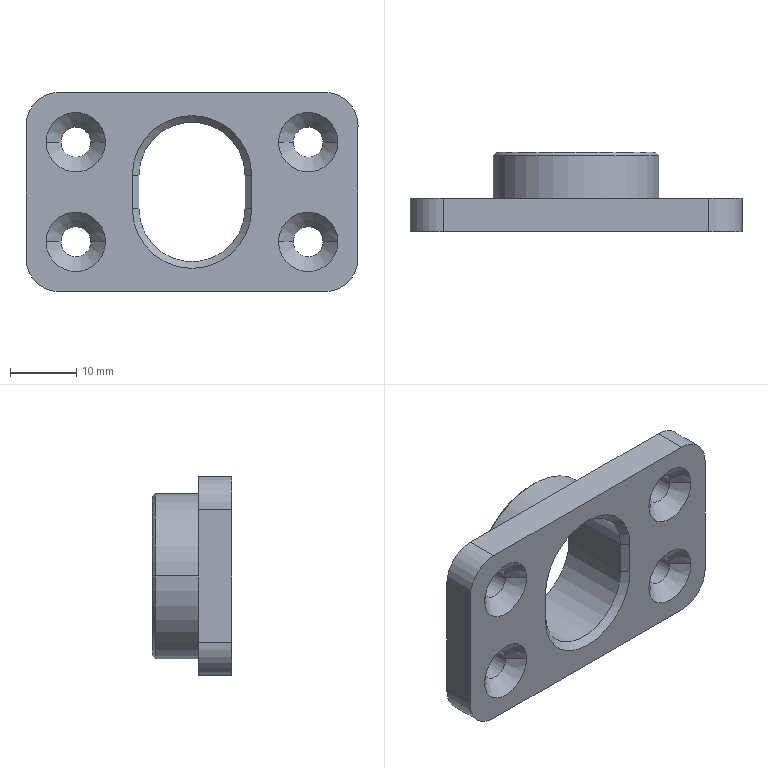Component | SolidWorks | MA060.03.03-08-1 | 1 solid | 39 faces | box 50 x 12 x 30 mm | volume 6910 mm3 | cylinder 16 | cone 12 | plane 11 | commonest cylinder face diameters 4.5 x8 10 x4 25 x2 16 x2 | material H68
build123d program:
from build123d import *

# Parameters (mm, degrees)
SKETCH1_W                                            = 50
SKETCH1_H                                            = 30
BOSS_EXTRUDE1_DEPTH                                  = 5
SKETCH2_R                                            = 12.5
BOSS_EXTRUDE2_DEPTH                                  = 7
CUT_EXTRUDE1_DEPTH                                   = 32.528
FILLET1_R                                            = 5
CHAMFER1_SIZE                                        = 0.5
CHAMFER2_SIZE                                        = 1
M4_CONICAL_COUNTERSUNK_HOLE_FOR_HEX_SOCK_D           = 4.5
M4_CONICAL_COUNTERSUNK_HOLE_FOR_HEX_SOCK_CSINK_D     = 8.96
M4_CONICAL_COUNTERSUNK_HOLE_FOR_HEX_SOCK_CSINK_ANGLE = 90
LPATTERN1_COUNT                                      = 2
LPATTERN1_PITCH                                      = 15
LPATTERN1_COUNT_DIR2                                 = 2
LPATTERN1_PITCH_DIR2                                 = 35


with BuildPart() as part:
    # Sketch1 → Boss-Extrude1 (new body)
    with BuildSketch(Plane.XY):
        Rectangle(SKETCH1_W, SKETCH1_H)
    extrude(amount=BOSS_EXTRUDE1_DEPTH)

    # Sketch2 → Boss-Extrude2 (add)
    with BuildSketch(Plane.XY.offset(5)):
        with Locations(Location((0, 0, 0), (0, 0, 180))):
            Circle(SKETCH2_R)
    extrude(amount=BOSS_EXTRUDE2_DEPTH)

    # Sketch3 → Cut-Extrude1 (cut, through all)
    with BuildSketch(Plane.XY.offset(12)):
        with BuildLine():
            Line((-8, -2.5), (-8, 2.5))
            ThreePointArc((-8, 2.5), (0, 10.5), (8, 2.5))
            Line((8, 2.5), (8, -2.5))
            ThreePointArc((8, -2.5), (0, -10.5), (-8, -2.5))
        make_face()
    extrude(amount=-CUT_EXTRUDE1_DEPTH, mode=Mode.SUBTRACT)

    # Fillet1
    fillet1_edges = [part.edges().sort_by_distance(p)[0] for p in [
        (25, -15, 2.5),
        (-25, -15, 2.5),
        (-25, 15, 2.5),
        (25, 15, 2.5),
    ]]
    fillet(fillet1_edges, radius=FILLET1_R)

    # Chamfer1
    chamfer1_edges = [part.edges().sort_by_distance(p)[0] for p in [
        (12.5, 0, 12),
    ]]
    chamfer(chamfer1_edges, length=CHAMFER1_SIZE)

    # Chamfer2
    chamfer2_edges = [part.edges().sort_by_distance(p)[0] for p in [
        (0, -10.5, 0),
        (-8, 0, 0),
        (0, 10.5, 0),
        (8, 0, 0),
    ]]
    chamfer(chamfer2_edges, length=CHAMFER2_SIZE)

    # M4 Conical Countersunk Hole for Hex Sock (through all)
    with Locations(Plane(origin=(0, 0, 0), x_dir=(-1, 0, 0), z_dir=(0, 0, -1))):
        with Locations((17.5, -7.5)):
            m4_conical_countersunk_hole_for_hex_sock = CounterSinkHole(M4_CONICAL_COUNTERSUNK_HOLE_FOR_HEX_SOCK_D / 2, M4_CONICAL_COUNTERSUNK_HOLE_FOR_HEX_SOCK_CSINK_D / 2, counter_sink_angle=M4_CONICAL_COUNTERSUNK_HOLE_FOR_HEX_SOCK_CSINK_ANGLE)

    # LPattern1: M4 Conical Countersunk Hole for Hex Sock 2 × 2
    with Locations(*[(j * LPATTERN1_PITCH_DIR2, i * LPATTERN1_PITCH, 0) for i in range(LPATTERN1_COUNT) for j in range(LPATTERN1_COUNT_DIR2) if (i, j) != (0, 0)]):
        add(m4_conical_countersunk_hole_for_hex_sock, mode=Mode.SUBTRACT)


solid = part.part

# Placed as in the assembly
solid = solid.moved(Location((0, 78.053, -99), (-90, 0, 0)))